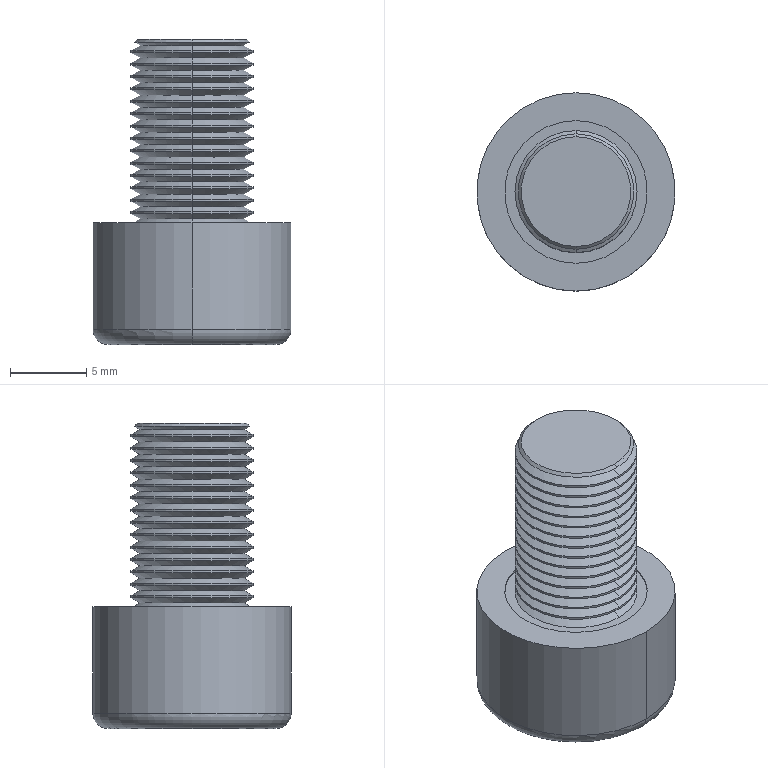Component | SolidWorks | LongSideClampingAssemblyBGeneralAssembly-1_HexagonSocketHeadCapScrew-M8X12-0510-1 | 1 solid | 114 faces | box 13 x 13 x 20 mm | volume 1442 mm3 | cone 64 | cylinder 32 | plane 16 | torus 2 | commonest cylinder face diameters 8 x28 13 x2 9.353 x2
build123d program:
from build123d import *

# Parameters (mm, degrees)
SKETCH1_R           = 6.5
BASEHEAD_DEPTH      = 8
SKETCH2_R           = 4
BASEBODY_DEPTH      = 12
HEXAGONSOCKET_DEPTH = 4
TOPFILLET_R         = 1
CHAMFER1_SIZE       = 0.4
LPATTERN10_COUNT    = 15
LPATTERN10_PITCH    = 0.8118


with BuildPart() as part:
    # Sketch1 → BaseHead (new body)
    with BuildSketch(Plane(origin=(0, 0, 0), x_dir=(0, 0, -1), z_dir=(1, 0, 0))):
        Circle(SKETCH1_R)
    extrude(amount=BASEHEAD_DEPTH)

    # Sketch2 → BaseBody (add)
    with BuildSketch(Plane(origin=(8, 0, 0), x_dir=(0, 0, -1), z_dir=(1, 0, 0))):
        Circle(SKETCH2_R)
    extrude(amount=BASEBODY_DEPTH)

    # Sketch3 → HexagonSocket (cut)
    with BuildSketch(Plane(origin=(0, 0, 0), x_dir=(0, 0, -1), z_dir=(1, 0, 0))):
        Polygon((3.464, 0), (1.732, 3), (-1.732, 3), (-3.464, 0), (-1.732, -3), (1.732, -3), align=None)
    extrude(amount=HEXAGONSOCKET_DEPTH, mode=Mode.SUBTRACT)

    # Sketch4 → Cut-Revolve1 (revolve, cut)
    with BuildSketch(Plane(origin=(-4.196, 0.75, 0), x_dir=(-1, 0, 0), z_dir=(0, 0, 1)), mode=Mode.PRIVATE) as cut_revolve1_sk:
        Polygon((-8.196, 3.75), (-9.928, 0.75), (-8.196, 0.75), align=None)
    revolve(cut_revolve1_sk.sketch.rotate(Axis((0.839, 0, 0), (-1, 0, 0)), 90), axis=Axis((0.839, 0, 0), (-1, 0, 0)), mode=Mode.SUBTRACT)

    # TopFillet
    topfillet_edges = [part.edges().sort_by_distance(p)[0] for p in [
        (0, 0, 6.5),
    ]]
    fillet(topfillet_edges, radius=TOPFILLET_R)

    # Chamfer1
    chamfer1_edges = [part.edges().sort_by_distance(p)[0] for p in [
        (20, 0, 4),
    ]]
    chamfer(chamfer1_edges, length=CHAMFER1_SIZE)

    # Sketch5 → Cut-Revolve10 (revolve, cut)
    with BuildSketch(Plane.XY, mode=Mode.PRIVATE) as cut_revolve10_sk:
        Polygon((19.6, 3.414), (19.938, 4), (19.938, 4.676), (19.262, 4.676), (19.262, 4), align=None)
    cut_revolve10 = revolve(cut_revolve10_sk.sketch.rotate(Axis((0, 0, 0), (1, 0, 0)), 90), axis=Axis((0, 0, 0), (1, 0, 0)), mode=Mode.SUBTRACT)

    # LPattern10: Cut-Revolve10 ×15
    with Locations(*[(-i * LPATTERN10_PITCH, 0, 0) for i in range(1, LPATTERN10_COUNT)]):
        add(cut_revolve10, mode=Mode.SUBTRACT)


solid = part.part

# Placed as in the assembly
solid = solid.moved(Location((-3191.658, -19.609, 3487.5), (90, 0, 90)))